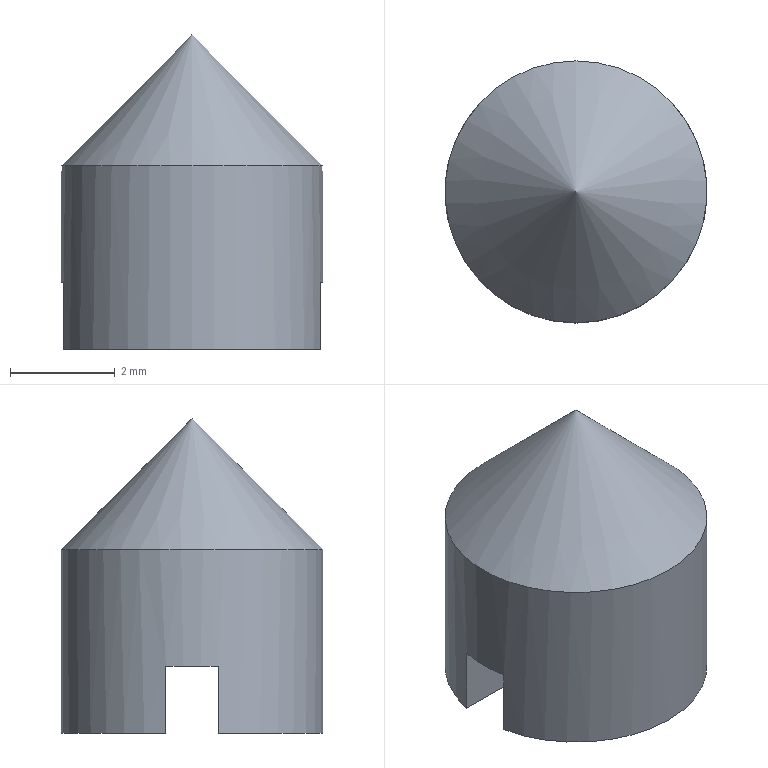Component | NX | M5X6 | 1 solid | 7 faces | box 5 x 5 x 6 mm | volume 79 mm3 | plane 5 | cylinder 1 | cone 1 | commonest cylinder face diameters 5 x1
STEP:
#1=CARTESIAN_POINT('',(0.,0.,0.));
#2=DIRECTION('',(0.,0.,1.));
#3=DIRECTION('',(1.,0.,0.));
#4=AXIS2_PLACEMENT_3D('',#1,#2,#3);
#5=CARTESIAN_POINT('',(-42.449,-34.,85.957));
#6=VERTEX_POINT('',#5);
#7=CARTESIAN_POINT('',(-37.551,-34.,85.957));
#8=VERTEX_POINT('',#7);
#9=CARTESIAN_POINT('',(-43.233,-34.,85.957));
#10=DIRECTION('',(1.,0.,0.));
#11=VECTOR('',#10,1.);
#12=LINE('',#9,#11);
#13=CARTESIAN_POINT('',(-40.,-37.,85.957));
#14=DIRECTION('',(0.,-0.,-1.));
#15=DIRECTION('',(0.,1.,-0.));
#16=AXIS2_PLACEMENT_3D('',#13,#14,#15);
#17=PLANE('',#16);
#18=CARTESIAN_POINT('',(3.,-3.233));
#19=DIRECTION('',(0.,1.));
#20=VECTOR('',#19,1.);
#21=LINE('',#18,#20);
#22=(GEOMETRIC_REPRESENTATION_CONTEXT(2)PARAMETRIC_REPRESENTATION_CONTEXT()REPRESENTATION_CONTEXT('',''));
#23=DEFINITIONAL_REPRESENTATION('',(#21),#22);
#24=PCURVE('',#17,#23);
#25=CARTESIAN_POINT('',(-43.233,-34.,87.237));
#26=DIRECTION('',(-0.,1.,0.));
#27=DIRECTION('',(1.,0.,0.));
#28=AXIS2_PLACEMENT_3D('',#25,#26,#27);
#29=PLANE('',#28);
#30=CARTESIAN_POINT('',(0.,1.28));
#31=DIRECTION('',(1.,0.));
#32=VECTOR('',#31,1.);
#33=LINE('',#30,#32);
#34=(GEOMETRIC_REPRESENTATION_CONTEXT(2)PARAMETRIC_REPRESENTATION_CONTEXT()REPRESENTATION_CONTEXT('',''));
#35=DEFINITIONAL_REPRESENTATION('',(#33),#34);
#36=PCURVE('',#29,#35);
#37=SURFACE_CURVE('',#12,(#24,#36),.PCURVE_S1.);
#38=EDGE_CURVE('',#6,#8,#37,.T.);
#39=ORIENTED_EDGE('',*,*,#38,.F.);
#40=CARTESIAN_POINT('',(-40.,-34.5,85.957));
#41=DIRECTION('',(0.,0.,1.));
#42=DIRECTION('',(0.,-1.,0.));
#43=AXIS2_PLACEMENT_3D('',#40,#41,#42);
#44=CIRCLE('',#43,2.5);
#45=CARTESIAN_POINT('',(0.,0.));
#46=CARTESIAN_POINT('',(0.,4.33));
#47=CARTESIAN_POINT('',(3.75,2.165));
#48=CARTESIAN_POINT('',(7.5,0.));
#49=CARTESIAN_POINT('',(3.75,-2.165));
#50=CARTESIAN_POINT('',(0.,-4.33));
#51=CARTESIAN_POINT('',(0.,0.));
#52=(BOUNDED_CURVE()B_SPLINE_CURVE(2,(#45,#46,#47,#48,#49,#50,#51),.UNSPECIFIED.,.T.,.F.)B_SPLINE_CURVE_WITH_KNOTS((1,2,2,2,2,1),(-2.094,0.,2.094,4.189,6.283,8.378),.UNSPECIFIED.)CURVE()GEOMETRIC_REPRESENTATION_ITEM()RATIONAL_B_SPLINE_CURVE((1.,0.5,1.,0.5,1.,0.5,1.))REPRESENTATION_ITEM(''));
#53=(GEOMETRIC_REPRESENTATION_CONTEXT(2)PARAMETRIC_REPRESENTATION_CONTEXT()REPRESENTATION_CONTEXT('',''));
#54=DEFINITIONAL_REPRESENTATION('',(#52),#53);
#55=PCURVE('',#17,#54);
#56=CARTESIAN_POINT('',(-40.,-34.5,85.957));
#57=DIRECTION('',(0.,0.,1.));
#58=DIRECTION('',(0.,-1.,0.));
#59=AXIS2_PLACEMENT_3D('',#56,#57,#58);
#60=CYLINDRICAL_SURFACE('',#59,2.5);
#61=CARTESIAN_POINT('',(0.,0.));
#62=DIRECTION('',(1.,0.));
#63=VECTOR('',#62,1.);
#64=LINE('',#61,#63);
#65=(GEOMETRIC_REPRESENTATION_CONTEXT(2)PARAMETRIC_REPRESENTATION_CONTEXT()REPRESENTATION_CONTEXT('',''));
#66=DEFINITIONAL_REPRESENTATION('',(#64),#65);
#67=PCURVE('',#60,#66);
#68=SURFACE_CURVE('',#44,(#55,#67),.PCURVE_S1.);
#69=EDGE_CURVE('',#8,#6,#68,.T.);
#70=ORIENTED_EDGE('',*,*,#69,.F.);
#71=EDGE_LOOP('',(#39,#70));
#72=FACE_BOUND('',#71,.T.);
#73=ADVANCED_FACE('',(#72),#17,.T.);
#74=CARTESIAN_POINT('',(-42.449,-34.,87.237));
#75=VERTEX_POINT('',#74);
#76=CARTESIAN_POINT('',(-42.449,-34.,85.957));
#77=DIRECTION('',(0.,-0.,-1.));
#78=VECTOR('',#77,1.);
#79=LINE('',#76,#78);
#80=CARTESIAN_POINT('',(4.511,0.));
#81=DIRECTION('',(0.,-1.));
#82=VECTOR('',#81,1.);
#83=LINE('',#80,#82);
#84=(GEOMETRIC_REPRESENTATION_CONTEXT(2)PARAMETRIC_REPRESENTATION_CONTEXT()REPRESENTATION_CONTEXT('',''));
#85=DEFINITIONAL_REPRESENTATION('',(#83),#84);
#86=PCURVE('',#60,#85);
#87=CARTESIAN_POINT('',(0.7831,1.28));
#88=DIRECTION('',(-0.,1.));
#89=VECTOR('',#88,1.);
#90=LINE('',#87,#89);
#91=(GEOMETRIC_REPRESENTATION_CONTEXT(2)PARAMETRIC_REPRESENTATION_CONTEXT()REPRESENTATION_CONTEXT('',''));
#92=DEFINITIONAL_REPRESENTATION('',(#90),#91);
#93=PCURVE('',#29,#92);
#94=SURFACE_CURVE('',#79,(#86,#93),.PCURVE_S1.);
#95=EDGE_CURVE('',#75,#6,#94,.T.);
#96=ORIENTED_EDGE('',*,*,#95,.F.);
#97=CARTESIAN_POINT('',(-42.449,-35.,87.237));
#98=VERTEX_POINT('',#97);
#99=CARTESIAN_POINT('',(-40.,-34.5,87.237));
#100=DIRECTION('',(0.,0.,1.));
#101=DIRECTION('',(1.,0.,0.));
#102=AXIS2_PLACEMENT_3D('',#99,#100,#101);
#103=CIRCLE('',#102,2.5);
#104=CARTESIAN_POINT('',(1.571,1.28));
#105=DIRECTION('',(1.,0.));
#106=VECTOR('',#105,1.);
#107=LINE('',#104,#106);
#108=(GEOMETRIC_REPRESENTATION_CONTEXT(2)PARAMETRIC_REPRESENTATION_CONTEXT()REPRESENTATION_CONTEXT('',''));
#109=DEFINITIONAL_REPRESENTATION('',(#107),#108);
#110=PCURVE('',#60,#109);
#111=CARTESIAN_POINT('',(-40.,-34.5,87.237));
#112=DIRECTION('',(0.,0.,-1.));
#113=DIRECTION('',(1.,0.,0.));
#114=AXIS2_PLACEMENT_3D('',#111,#112,#113);
#115=PLANE('',#114);
#116=CARTESIAN_POINT('',(2.5,0.));
#117=CARTESIAN_POINT('',(2.5,-4.33));
#118=CARTESIAN_POINT('',(-1.25,-2.165));
#119=CARTESIAN_POINT('',(-5.,-0.));
#120=CARTESIAN_POINT('',(-1.25,2.165));
#121=CARTESIAN_POINT('',(2.5,4.33));
#122=CARTESIAN_POINT('',(2.5,0.));
#123=(BOUNDED_CURVE()B_SPLINE_CURVE(2,(#116,#117,#118,#119,#120,#121,#122),.UNSPECIFIED.,.T.,.F.)B_SPLINE_CURVE_WITH_KNOTS((1,2,2,2,2,1),(-2.094,0.,2.094,4.189,6.283,8.378),.UNSPECIFIED.)CURVE()GEOMETRIC_REPRESENTATION_ITEM()RATIONAL_B_SPLINE_CURVE((1.,0.5,1.,0.5,1.,0.5,1.))REPRESENTATION_ITEM(''));
#124=(GEOMETRIC_REPRESENTATION_CONTEXT(2)PARAMETRIC_REPRESENTATION_CONTEXT()REPRESENTATION_CONTEXT('',''));
#125=DEFINITIONAL_REPRESENTATION('',(#123),#124);
#126=PCURVE('',#115,#125);
#127=SURFACE_CURVE('',#103,(#110,#126),.PCURVE_S1.);
#128=EDGE_CURVE('',#75,#98,#127,.T.);
#129=ORIENTED_EDGE('',*,*,#128,.T.);
#130=CARTESIAN_POINT('',(-42.449,-35.,85.957));
#131=VERTEX_POINT('',#130);
#132=CARTESIAN_POINT('',(-42.449,-35.,85.957));
#133=DIRECTION('',(0.,0.,1.));
#134=VECTOR('',#133,1.);
#135=LINE('',#132,#134);
#136=CARTESIAN_POINT('',(4.914,0.));
#137=DIRECTION('',(0.,1.));
#138=VECTOR('',#137,1.);
#139=LINE('',#136,#138);
#140=(GEOMETRIC_REPRESENTATION_CONTEXT(2)PARAMETRIC_REPRESENTATION_CONTEXT()REPRESENTATION_CONTEXT('',''));
#141=DEFINITIONAL_REPRESENTATION('',(#139),#140);
#142=PCURVE('',#60,#141);
#143=CARTESIAN_POINT('',(-37.045,-35.,87.237));
#144=DIRECTION('',(0.,-1.,0.));
#145=DIRECTION('',(0.,0.,-1.));
#146=AXIS2_PLACEMENT_3D('',#143,#144,#145);
#147=PLANE('',#146);
#148=CARTESIAN_POINT('',(1.28,-5.405));
#149=DIRECTION('',(-1.,0.));
#150=VECTOR('',#149,1.);
#151=LINE('',#148,#150);
#152=(GEOMETRIC_REPRESENTATION_CONTEXT(2)PARAMETRIC_REPRESENTATION_CONTEXT()REPRESENTATION_CONTEXT('',''));
#153=DEFINITIONAL_REPRESENTATION('',(#151),#152);
#154=PCURVE('',#147,#153);
#155=SURFACE_CURVE('',#135,(#142,#154),.PCURVE_S1.);
#156=EDGE_CURVE('',#131,#98,#155,.T.);
#157=ORIENTED_EDGE('',*,*,#156,.F.);
#158=CARTESIAN_POINT('',(-40.,-37.,85.957));
#159=VERTEX_POINT('',#158);
#160=CARTESIAN_POINT('',(-40.,-34.5,85.957));
#161=DIRECTION('',(0.,0.,1.));
#162=DIRECTION('',(0.,-1.,0.));
#163=AXIS2_PLACEMENT_3D('',#160,#161,#162);
#164=CIRCLE('',#163,2.5);
#165=CARTESIAN_POINT('',(-0.,0.));
#166=DIRECTION('',(1.,0.));
#167=VECTOR('',#166,1.);
#168=LINE('',#165,#167);
#169=(GEOMETRIC_REPRESENTATION_CONTEXT(2)PARAMETRIC_REPRESENTATION_CONTEXT()REPRESENTATION_CONTEXT('',''));
#170=DEFINITIONAL_REPRESENTATION('',(#168),#169);
#171=PCURVE('',#60,#170);
#172=CARTESIAN_POINT('',(-40.,-37.,85.957));
#173=DIRECTION('',(0.,-0.,-1.));
#174=DIRECTION('',(0.,1.,-0.));
#175=AXIS2_PLACEMENT_3D('',#172,#173,#174);
#176=PLANE('',#175);
#177=CARTESIAN_POINT('',(0.,0.));
#178=CARTESIAN_POINT('',(0.,4.33));
#179=CARTESIAN_POINT('',(3.75,2.165));
#180=CARTESIAN_POINT('',(7.5,0.));
#181=CARTESIAN_POINT('',(3.75,-2.165));
#182=CARTESIAN_POINT('',(0.,-4.33));
#183=CARTESIAN_POINT('',(0.,0.));
#184=(BOUNDED_CURVE()B_SPLINE_CURVE(2,(#177,#178,#179,#180,#181,#182,#183),.UNSPECIFIED.,.T.,.F.)B_SPLINE_CURVE_WITH_KNOTS((1,2,2,2,2,1),(-2.094,0.,2.094,4.189,6.283,8.378),.UNSPECIFIED.)CURVE()GEOMETRIC_REPRESENTATION_ITEM()RATIONAL_B_SPLINE_CURVE((1.,0.5,1.,0.5,1.,0.5,1.))REPRESENTATION_ITEM(''));
#185=(GEOMETRIC_REPRESENTATION_CONTEXT(2)PARAMETRIC_REPRESENTATION_CONTEXT()REPRESENTATION_CONTEXT('',''));
#186=DEFINITIONAL_REPRESENTATION('',(#184),#185);
#187=PCURVE('',#176,#186);
#188=SURFACE_CURVE('',#164,(#171,#187),.PCURVE_S1.);
#189=EDGE_CURVE('',#131,#159,#188,.T.);
#190=ORIENTED_EDGE('',*,*,#189,.T.);
#191=CARTESIAN_POINT('',(-40.,-37.,89.457));
#192=VERTEX_POINT('',#191);
#193=CARTESIAN_POINT('',(-40.,-37.,85.957));
#194=CARTESIAN_POINT('',(-40.,-37.,89.457));
#195=B_SPLINE_CURVE_WITH_KNOTS('',1,(#193,#194),.UNSPECIFIED.,.F.,.F.,(2,2),(0.,3.5),.PIECEWISE_BEZIER_KNOTS.);
#196=CARTESIAN_POINT('',(6.283,0.));
#197=DIRECTION('',(0.,1.));
#198=VECTOR('',#197,1.);
#199=LINE('',#196,#198);
#200=(GEOMETRIC_REPRESENTATION_CONTEXT(2)PARAMETRIC_REPRESENTATION_CONTEXT()REPRESENTATION_CONTEXT('',''));
#201=DEFINITIONAL_REPRESENTATION('',(#199),#200);
#202=PCURVE('',#60,#201);
#203=CARTESIAN_POINT('',(0.,0.));
#204=DIRECTION('',(0.,1.));
#205=VECTOR('',#204,1.);
#206=LINE('',#203,#205);
#207=(GEOMETRIC_REPRESENTATION_CONTEXT(2)PARAMETRIC_REPRESENTATION_CONTEXT()REPRESENTATION_CONTEXT('',''));
#208=DEFINITIONAL_REPRESENTATION('',(#206),#207);
#209=PCURVE('',#60,#208);
#210=SEAM_CURVE('',#195,(#202,#209),.PCURVE_S1.);
#211=EDGE_CURVE('',#159,#192,#210,.T.);
#212=ORIENTED_EDGE('',*,*,#211,.T.);
#213=CARTESIAN_POINT('',(-40.,-32.,89.457));
#214=VERTEX_POINT('',#213);
#215=CARTESIAN_POINT('',(-40.,-34.5,89.457));
#216=DIRECTION('',(0.,0.,1.));
#217=DIRECTION('',(0.,-1.,0.));
#218=AXIS2_PLACEMENT_3D('',#215,#216,#217);
#219=CIRCLE('',#218,2.5);
#220=CARTESIAN_POINT('',(0.,3.5));
#221=DIRECTION('',(1.,0.));
#222=VECTOR('',#221,1.);
#223=LINE('',#220,#222);
#224=(GEOMETRIC_REPRESENTATION_CONTEXT(2)PARAMETRIC_REPRESENTATION_CONTEXT()REPRESENTATION_CONTEXT('',''));
#225=DEFINITIONAL_REPRESENTATION('',(#223),#224);
#226=PCURVE('',#60,#225);
#227=CARTESIAN_POINT('',(-40.,-34.5,91.957));
#228=DIRECTION('',(0.,-0.,-1.));
#229=DIRECTION('',(0.,1.,-0.));
#230=AXIS2_PLACEMENT_3D('',#227,#228,#229);
#231=CONICAL_SURFACE('',#230,0.,0.7854);
#232=CARTESIAN_POINT('',(9.425,2.5));
#233=DIRECTION('',(-1.,0.));
#234=VECTOR('',#233,1.);
#235=LINE('',#232,#234);
#236=(GEOMETRIC_REPRESENTATION_CONTEXT(2)PARAMETRIC_REPRESENTATION_CONTEXT()REPRESENTATION_CONTEXT('',''));
#237=DEFINITIONAL_REPRESENTATION('',(#235),#236);
#238=PCURVE('',#231,#237);
#239=SURFACE_CURVE('',#219,(#226,#238),.PCURVE_S1.);
#240=EDGE_CURVE('',#214,#192,#239,.T.);
#241=ORIENTED_EDGE('',*,*,#240,.F.);
#242=CARTESIAN_POINT('',(-40.,-34.5,89.457));
#243=DIRECTION('',(0.,0.,1.));
#244=DIRECTION('',(0.,-1.,0.));
#245=AXIS2_PLACEMENT_3D('',#242,#243,#244);
#246=CIRCLE('',#245,2.5);
#247=CARTESIAN_POINT('',(0.,3.5));
#248=DIRECTION('',(1.,0.));
#249=VECTOR('',#248,1.);
#250=LINE('',#247,#249);
#251=(GEOMETRIC_REPRESENTATION_CONTEXT(2)PARAMETRIC_REPRESENTATION_CONTEXT()REPRESENTATION_CONTEXT('',''));
#252=DEFINITIONAL_REPRESENTATION('',(#250),#251);
#253=PCURVE('',#60,#252);
#254=CARTESIAN_POINT('',(3.142,2.5));
#255=DIRECTION('',(-1.,0.));
#256=VECTOR('',#255,1.);
#257=LINE('',#254,#256);
#258=(GEOMETRIC_REPRESENTATION_CONTEXT(2)PARAMETRIC_REPRESENTATION_CONTEXT()REPRESENTATION_CONTEXT('',''));
#259=DEFINITIONAL_REPRESENTATION('',(#257),#258);
#260=PCURVE('',#231,#259);
#261=SURFACE_CURVE('',#246,(#253,#260),.PCURVE_S1.);
#262=EDGE_CURVE('',#192,#214,#261,.T.);
#263=ORIENTED_EDGE('',*,*,#262,.F.);
#264=ORIENTED_EDGE('',*,*,#211,.F.);
#265=CARTESIAN_POINT('',(-37.551,-35.,85.957));
#266=VERTEX_POINT('',#265);
#267=CARTESIAN_POINT('',(-40.,-34.5,85.957));
#268=DIRECTION('',(0.,0.,1.));
#269=DIRECTION('',(0.,-1.,0.));
#270=AXIS2_PLACEMENT_3D('',#267,#268,#269);
#271=CIRCLE('',#270,2.5);
#272=CARTESIAN_POINT('',(-0.,0.));
#273=DIRECTION('',(1.,0.));
#274=VECTOR('',#273,1.);
#275=LINE('',#272,#274);
#276=(GEOMETRIC_REPRESENTATION_CONTEXT(2)PARAMETRIC_REPRESENTATION_CONTEXT()REPRESENTATION_CONTEXT('',''));
#277=DEFINITIONAL_REPRESENTATION('',(#275),#276);
#278=PCURVE('',#60,#277);
#279=CARTESIAN_POINT('',(0.,0.));
#280=CARTESIAN_POINT('',(0.,4.33));
#281=CARTESIAN_POINT('',(3.75,2.165));
#282=CARTESIAN_POINT('',(7.5,0.));
#283=CARTESIAN_POINT('',(3.75,-2.165));
#284=CARTESIAN_POINT('',(0.,-4.33));
#285=CARTESIAN_POINT('',(0.,0.));
#286=(BOUNDED_CURVE()B_SPLINE_CURVE(2,(#279,#280,#281,#282,#283,#284,#285),.UNSPECIFIED.,.T.,.F.)B_SPLINE_CURVE_WITH_KNOTS((1,2,2,2,2,1),(-2.094,0.,2.094,4.189,6.283,8.378),.UNSPECIFIED.)CURVE()GEOMETRIC_REPRESENTATION_ITEM()RATIONAL_B_SPLINE_CURVE((1.,0.5,1.,0.5,1.,0.5,1.))REPRESENTATION_ITEM(''));
#287=(GEOMETRIC_REPRESENTATION_CONTEXT(2)PARAMETRIC_REPRESENTATION_CONTEXT()REPRESENTATION_CONTEXT('',''));
#288=DEFINITIONAL_REPRESENTATION('',(#286),#287);
#289=PCURVE('',#176,#288);
#290=SURFACE_CURVE('',#271,(#278,#289),.PCURVE_S1.);
#291=EDGE_CURVE('',#159,#266,#290,.T.);
#292=ORIENTED_EDGE('',*,*,#291,.T.);
#293=CARTESIAN_POINT('',(-37.551,-35.,87.237));
#294=VERTEX_POINT('',#293);
#295=CARTESIAN_POINT('',(-37.551,-35.,85.957));
#296=DIRECTION('',(0.,-0.,-1.));
#297=VECTOR('',#296,1.);
#298=LINE('',#295,#297);
#299=CARTESIAN_POINT('',(1.369,0.));
#300=DIRECTION('',(0.,-1.));
#301=VECTOR('',#300,1.);
#302=LINE('',#299,#301);
#303=(GEOMETRIC_REPRESENTATION_CONTEXT(2)PARAMETRIC_REPRESENTATION_CONTEXT()REPRESENTATION_CONTEXT('',''));
#304=DEFINITIONAL_REPRESENTATION('',(#302),#303);
#305=PCURVE('',#60,#304);
#306=CARTESIAN_POINT('',(1.28,-0.5056));
#307=DIRECTION('',(1.,0.));
#308=VECTOR('',#307,1.);
#309=LINE('',#306,#308);
#310=(GEOMETRIC_REPRESENTATION_CONTEXT(2)PARAMETRIC_REPRESENTATION_CONTEXT()REPRESENTATION_CONTEXT('',''));
#311=DEFINITIONAL_REPRESENTATION('',(#309),#310);
#312=PCURVE('',#147,#311);
#313=SURFACE_CURVE('',#298,(#305,#312),.PCURVE_S1.);
#314=EDGE_CURVE('',#294,#266,#313,.T.);
#315=ORIENTED_EDGE('',*,*,#314,.F.);
#316=CARTESIAN_POINT('',(-37.551,-34.,87.237));
#317=VERTEX_POINT('',#316);
#318=CARTESIAN_POINT('',(-40.,-34.5,87.237));
#319=DIRECTION('',(0.,0.,1.));
#320=DIRECTION('',(1.,0.,0.));
#321=AXIS2_PLACEMENT_3D('',#318,#319,#320);
#322=CIRCLE('',#321,2.5);
#323=CARTESIAN_POINT('',(-4.712,1.28));
#324=DIRECTION('',(1.,0.));
#325=VECTOR('',#324,1.);
#326=LINE('',#323,#325);
#327=(GEOMETRIC_REPRESENTATION_CONTEXT(2)PARAMETRIC_REPRESENTATION_CONTEXT()REPRESENTATION_CONTEXT('',''));
#328=DEFINITIONAL_REPRESENTATION('',(#326),#327);
#329=PCURVE('',#60,#328);
#330=CARTESIAN_POINT('',(2.5,0.));
#331=CARTESIAN_POINT('',(2.5,-4.33));
#332=CARTESIAN_POINT('',(-1.25,-2.165));
#333=CARTESIAN_POINT('',(-5.,-0.));
#334=CARTESIAN_POINT('',(-1.25,2.165));
#335=CARTESIAN_POINT('',(2.5,4.33));
#336=CARTESIAN_POINT('',(2.5,0.));
#337=(BOUNDED_CURVE()B_SPLINE_CURVE(2,(#330,#331,#332,#333,#334,#335,#336),.UNSPECIFIED.,.T.,.F.)B_SPLINE_CURVE_WITH_KNOTS((1,2,2,2,2,1),(-2.094,0.,2.094,4.189,6.283,8.378),.UNSPECIFIED.)CURVE()GEOMETRIC_REPRESENTATION_ITEM()RATIONAL_B_SPLINE_CURVE((1.,0.5,1.,0.5,1.,0.5,1.))REPRESENTATION_ITEM(''));
#338=(GEOMETRIC_REPRESENTATION_CONTEXT(2)PARAMETRIC_REPRESENTATION_CONTEXT()REPRESENTATION_CONTEXT('',''));
#339=DEFINITIONAL_REPRESENTATION('',(#337),#338);
#340=PCURVE('',#115,#339);
#341=SURFACE_CURVE('',#322,(#329,#340),.PCURVE_S1.);
#342=EDGE_CURVE('',#294,#317,#341,.T.);
#343=ORIENTED_EDGE('',*,*,#342,.T.);
#344=CARTESIAN_POINT('',(-37.551,-34.,85.957));
#345=DIRECTION('',(0.,0.,1.));
#346=VECTOR('',#345,1.);
#347=LINE('',#344,#346);
#348=CARTESIAN_POINT('',(1.772,0.));
#349=DIRECTION('',(0.,1.));
#350=VECTOR('',#349,1.);
#351=LINE('',#348,#350);
#352=(GEOMETRIC_REPRESENTATION_CONTEXT(2)PARAMETRIC_REPRESENTATION_CONTEXT()REPRESENTATION_CONTEXT('',''));
#353=DEFINITIONAL_REPRESENTATION('',(#351),#352);
#354=PCURVE('',#60,#353);
#355=CARTESIAN_POINT('',(5.682,1.28));
#356=DIRECTION('',(0.,-1.));
#357=VECTOR('',#356,1.);
#358=LINE('',#355,#357);
#359=(GEOMETRIC_REPRESENTATION_CONTEXT(2)PARAMETRIC_REPRESENTATION_CONTEXT()REPRESENTATION_CONTEXT('',''));
#360=DEFINITIONAL_REPRESENTATION('',(#358),#359);
#361=PCURVE('',#29,#360);
#362=SURFACE_CURVE('',#347,(#354,#361),.PCURVE_S1.);
#363=EDGE_CURVE('',#8,#317,#362,.T.);
#364=ORIENTED_EDGE('',*,*,#363,.F.);
#365=ORIENTED_EDGE('',*,*,#69,.T.);
#366=EDGE_LOOP('',(#96,#129,#157,#190,#212,#241,#263,#264,#292,#315,#343,#364,#365));
#367=FACE_BOUND('',#366,.T.);
#368=ADVANCED_FACE('',(#367),#60,.T.);
#369=CARTESIAN_POINT('',(-37.045,-35.,85.957));
#370=DIRECTION('',(-1.,0.,0.));
#371=VECTOR('',#370,1.);
#372=LINE('',#369,#371);
#373=CARTESIAN_POINT('',(2.,2.955));
#374=DIRECTION('',(0.,-1.));
#375=VECTOR('',#374,1.);
#376=LINE('',#373,#375);
#377=(GEOMETRIC_REPRESENTATION_CONTEXT(2)PARAMETRIC_REPRESENTATION_CONTEXT()REPRESENTATION_CONTEXT('',''));
#378=DEFINITIONAL_REPRESENTATION('',(#376),#377);
#379=PCURVE('',#176,#378);
#380=CARTESIAN_POINT('',(1.28,0.));
#381=DIRECTION('',(0.,-1.));
#382=VECTOR('',#381,1.);
#383=LINE('',#380,#382);
#384=(GEOMETRIC_REPRESENTATION_CONTEXT(2)PARAMETRIC_REPRESENTATION_CONTEXT()REPRESENTATION_CONTEXT('',''));
#385=DEFINITIONAL_REPRESENTATION('',(#383),#384);
#386=PCURVE('',#147,#385);
#387=SURFACE_CURVE('',#372,(#379,#386),.PCURVE_S1.);
#388=EDGE_CURVE('',#266,#131,#387,.T.);
#389=ORIENTED_EDGE('',*,*,#388,.F.);
#390=ORIENTED_EDGE('',*,*,#291,.F.);
#391=ORIENTED_EDGE('',*,*,#189,.F.);
#392=EDGE_LOOP('',(#389,#390,#391));
#393=FACE_BOUND('',#392,.T.);
#394=ADVANCED_FACE('',(#393),#176,.T.);
#395=ORIENTED_EDGE('',*,*,#262,.T.);
#396=CARTESIAN_POINT('',(-40.,-34.5,91.957));
#397=VERTEX_POINT('',#396);
#398=CARTESIAN_POINT('',(-40.,-34.5,91.957));
#399=CARTESIAN_POINT('',(-40.,-32.,89.457));
#400=B_SPLINE_CURVE_WITH_KNOTS('',1,(#398,#399),.UNSPECIFIED.,.F.,.F.,(2,2),(0.,3.536),.PIECEWISE_BEZIER_KNOTS.);
#401=CARTESIAN_POINT('',(0.,0.));
#402=DIRECTION('',(0.,1.));
#403=VECTOR('',#402,1.);
#404=LINE('',#401,#403);
#405=(GEOMETRIC_REPRESENTATION_CONTEXT(2)PARAMETRIC_REPRESENTATION_CONTEXT()REPRESENTATION_CONTEXT('',''));
#406=DEFINITIONAL_REPRESENTATION('',(#404),#405);
#407=PCURVE('',#231,#406);
#408=CARTESIAN_POINT('',(6.283,0.));
#409=DIRECTION('',(0.,1.));
#410=VECTOR('',#409,1.);
#411=LINE('',#408,#410);
#412=(GEOMETRIC_REPRESENTATION_CONTEXT(2)PARAMETRIC_REPRESENTATION_CONTEXT()REPRESENTATION_CONTEXT('',''));
#413=DEFINITIONAL_REPRESENTATION('',(#411),#412);
#414=PCURVE('',#231,#413);
#415=SEAM_CURVE('',#400,(#407,#414),.PCURVE_S1.);
#416=EDGE_CURVE('',#397,#214,#415,.T.);
#417=ORIENTED_EDGE('',*,*,#416,.F.);
#418=ORIENTED_EDGE('',*,*,#416,.T.);
#419=ORIENTED_EDGE('',*,*,#240,.T.);
#420=EDGE_LOOP('',(#395,#417,#418,#419));
#421=FACE_BOUND('',#420,.T.);
#422=ADVANCED_FACE('',(#421),#231,.T.);
#423=ORIENTED_EDGE('',*,*,#95,.T.);
#424=ORIENTED_EDGE('',*,*,#38,.T.);
#425=ORIENTED_EDGE('',*,*,#363,.T.);
#426=CARTESIAN_POINT('',(-43.233,-34.,87.237));
#427=DIRECTION('',(-1.,-0.,0.));
#428=VECTOR('',#427,1.);
#429=LINE('',#426,#428);
#430=CARTESIAN_POINT('',(0.,0.));
#431=DIRECTION('',(-1.,0.));
#432=VECTOR('',#431,1.);
#433=LINE('',#430,#432);
#434=(GEOMETRIC_REPRESENTATION_CONTEXT(2)PARAMETRIC_REPRESENTATION_CONTEXT()REPRESENTATION_CONTEXT('',''));
#435=DEFINITIONAL_REPRESENTATION('',(#433),#434);
#436=PCURVE('',#29,#435);
#437=CARTESIAN_POINT('',(-3.233,-0.5));
#438=DIRECTION('',(-1.,0.));
#439=VECTOR('',#438,1.);
#440=LINE('',#437,#439);
#441=(GEOMETRIC_REPRESENTATION_CONTEXT(2)PARAMETRIC_REPRESENTATION_CONTEXT()REPRESENTATION_CONTEXT('',''));
#442=DEFINITIONAL_REPRESENTATION('',(#440),#441);
#443=PCURVE('',#115,#442);
#444=SURFACE_CURVE('',#429,(#436,#443),.PCURVE_S1.);
#445=EDGE_CURVE('',#317,#75,#444,.T.);
#446=ORIENTED_EDGE('',*,*,#445,.T.);
#447=EDGE_LOOP('',(#423,#424,#425,#446));
#448=FACE_BOUND('',#447,.T.);
#449=ADVANCED_FACE('',(#448),#29,.F.);
#450=ORIENTED_EDGE('',*,*,#314,.T.);
#451=ORIENTED_EDGE('',*,*,#388,.T.);
#452=ORIENTED_EDGE('',*,*,#156,.T.);
#453=CARTESIAN_POINT('',(-37.045,-35.,87.237));
#454=DIRECTION('',(1.,0.,0.));
#455=VECTOR('',#454,1.);
#456=LINE('',#453,#455);
#457=CARTESIAN_POINT('',(0.,0.));
#458=DIRECTION('',(0.,1.));
#459=VECTOR('',#458,1.);
#460=LINE('',#457,#459);
#461=(GEOMETRIC_REPRESENTATION_CONTEXT(2)PARAMETRIC_REPRESENTATION_CONTEXT()REPRESENTATION_CONTEXT('',''));
#462=DEFINITIONAL_REPRESENTATION('',(#460),#461);
#463=PCURVE('',#147,#462);
#464=CARTESIAN_POINT('',(2.955,0.5));
#465=DIRECTION('',(1.,0.));
#466=VECTOR('',#465,1.);
#467=LINE('',#464,#466);
#468=(GEOMETRIC_REPRESENTATION_CONTEXT(2)PARAMETRIC_REPRESENTATION_CONTEXT()REPRESENTATION_CONTEXT('',''));
#469=DEFINITIONAL_REPRESENTATION('',(#467),#468);
#470=PCURVE('',#115,#469);
#471=SURFACE_CURVE('',#456,(#463,#470),.PCURVE_S1.);
#472=EDGE_CURVE('',#98,#294,#471,.T.);
#473=ORIENTED_EDGE('',*,*,#472,.T.);
#474=EDGE_LOOP('',(#450,#451,#452,#473));
#475=FACE_BOUND('',#474,.T.);
#476=ADVANCED_FACE('',(#475),#147,.F.);
#477=ORIENTED_EDGE('',*,*,#445,.F.);
#478=ORIENTED_EDGE('',*,*,#342,.F.);
#479=ORIENTED_EDGE('',*,*,#472,.F.);
#480=ORIENTED_EDGE('',*,*,#128,.F.);
#481=EDGE_LOOP('',(#477,#478,#479,#480));
#482=FACE_BOUND('',#481,.T.);
#483=ADVANCED_FACE('',(#482),#115,.T.);
#484=CLOSED_SHELL('',(#73,#368,#394,#422,#449,#476,#483));
#485=MANIFOLD_SOLID_BREP('',#484);
#486=(LENGTH_UNIT()NAMED_UNIT(*)SI_UNIT(.MILLI.,.METRE.));
#487=UNCERTAINTY_MEASURE_WITH_UNIT(LENGTH_MEASURE(0.000002),#486,'','');
#488=(NAMED_UNIT(*)PLANE_ANGLE_UNIT()SI_UNIT($,.RADIAN.));
#489=(NAMED_UNIT(*)SI_UNIT($,.STERADIAN.)SOLID_ANGLE_UNIT());
#490=(GEOMETRIC_REPRESENTATION_CONTEXT(3)GLOBAL_UNCERTAINTY_ASSIGNED_CONTEXT((#487))GLOBAL_UNIT_ASSIGNED_CONTEXT((#486,#488,#489))REPRESENTATION_CONTEXT('',''));
#491=ADVANCED_BREP_SHAPE_REPRESENTATION('',(#4,#485),#490);